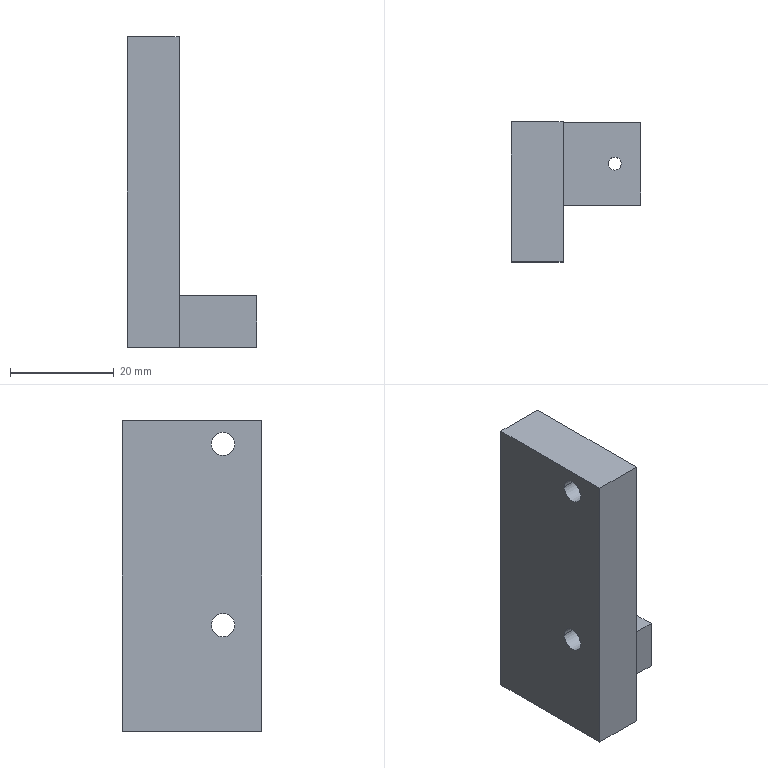Component | SolidWorks | F-YBExport-1-1_LSDH-6-026-1 | 1 solid | 21 faces | box 25 x 27 x 60 mm | volume 17917 mm3 | plane 11 | cylinder 10 | commonest cylinder face diameters 8 x4 4.5 x4 2.5 x2
build123d program:
from build123d import *

# Parameters (mm, degrees)
SKETCH1_W                                            = 60
SKETCH1_H                                            = 10
BOSS_EXTRUDE1_DEPTH                                  = 27
SKETCH2_W                                            = 10
SKETCH2_H                                            = 27
BOSS_EXTRUDE2_DEPTH                                  = 25
HOLE_SIZE_ACCORDING_TO_THE_TYPE_OF_HEX_S_D           = 4.5
HOLE_SIZE_ACCORDING_TO_THE_TYPE_OF_HEX_S_CBORE_D     = 8
HOLE_SIZE_ACCORDING_TO_THE_TYPE_OF_HEX_S_CBORE_DEPTH = 4.6
SKETCH5_W                                            = 11
SKETCH5_H                                            = 25
CUT_EXTRUDE1_DEPTH                                   = 73.312
M3_TAPPED_HOLE1_D                                    = 2.5
SKETCH8_W                                            = 16
SKETCH8_H                                            = 10
CUT_EXTRUDE2_DEPTH                                   = 65.257


with BuildPart() as part:
    # Sketch1 → Boss-Extrude1 (new body)
    with BuildSketch(Plane.XY):
        Rectangle(SKETCH1_W, SKETCH1_H)
    extrude(amount=BOSS_EXTRUDE1_DEPTH)

    # Sketch2 → Boss-Extrude2 (add)
    with BuildSketch(Plane.XZ.offset(5)):
        with Locations((25, 13.5)):
            Rectangle(SKETCH2_W, SKETCH2_H)
    extrude(amount=BOSS_EXTRUDE2_DEPTH)

    # Hole size according to the type of hex s (through all)
    with Locations(Plane(origin=(-25.5, -5, 7.5), x_dir=(0, 0, -1), z_dir=(0, -1, 0))):
        with Locations((0, 0), (0, 35)):
            CounterBoreHole(HOLE_SIZE_ACCORDING_TO_THE_TYPE_OF_HEX_S_D / 2, HOLE_SIZE_ACCORDING_TO_THE_TYPE_OF_HEX_S_CBORE_D / 2, HOLE_SIZE_ACCORDING_TO_THE_TYPE_OF_HEX_S_CBORE_DEPTH)

    # Sketch5 → Cut-Extrude1 (cut, through all)
    with BuildSketch(Plane(origin=(30, 0, 0), x_dir=(0, 0, -1), z_dir=(1, 0, 0))):
        with Locations((-5.5, -17.5)):
            Rectangle(SKETCH5_W, SKETCH5_H)
    extrude(amount=-CUT_EXTRUDE1_DEPTH, mode=Mode.SUBTRACT)

    # M3 Tapped Hole1 (through all)
    with Locations(Plane(origin=(20, -15, 19), x_dir=(0, 0, -1), z_dir=(-1, 0, 0))):
        with Locations((0, 0), (0, 10)):
            Hole(M3_TAPPED_HOLE1_D / 2)

    # Sketch8 → Cut-Extrude2 (cut, through all)
    with BuildSketch(Plane.ZY.offset(-20)):
        with Locations((19, -25)):
            Rectangle(SKETCH8_W, SKETCH8_H)
    extrude(amount=-CUT_EXTRUDE2_DEPTH, mode=Mode.SUBTRACT)


solid = part.part

# Placed as in the assembly
solid = solid.moved(Location((406.305, 356.175, 167.979), (-90, 0, 90)))
STEP:
#1=COLOUR_RGB('',0.7922,0.8196,0.9333);
#2=FILL_AREA_STYLE_COLOUR('',#1);
#3=FILL_AREA_STYLE('',(#2));
#4=SURFACE_STYLE_FILL_AREA(#3);
#5=SURFACE_SIDE_STYLE('',(#4));
#6=SURFACE_STYLE_USAGE(.BOTH.,#5);
#7=PRESENTATION_STYLE_ASSIGNMENT((#6));
#8=CARTESIAN_POINT('',(16.587,14.721,5.432));
#9=VERTEX_POINT('',#8);
#10=CARTESIAN_POINT('',(16.587,14.82,5.432));
#11=VERTEX_POINT('',#10);
#12=CARTESIAN_POINT('',(16.587,14.771,5.432));
#13=DIRECTION('',(-0.,-0.,1.));
#14=DIRECTION('',(0.,1.,0.));
#15=AXIS2_PLACEMENT_3D('',#12,#13,#14);
#16=CIRCLE('',#15,0.04921);
#17=EDGE_CURVE('',#9,#11,#16,.T.);
#18=ORIENTED_EDGE('',*,*,#17,.F.);
#19=CARTESIAN_POINT('',(16.587,14.721,5.826));
#20=VERTEX_POINT('',#19);
#21=CARTESIAN_POINT('',(16.587,14.721,5.826));
#22=DIRECTION('',(-0.,-0.,1.));
#23=VECTOR('',#22,39.37);
#24=LINE('',#21,#23);
#25=EDGE_CURVE('',#9,#20,#24,.T.);
#26=ORIENTED_EDGE('',*,*,#25,.T.);
#27=CARTESIAN_POINT('',(16.587,14.82,5.826));
#28=VERTEX_POINT('',#27);
#29=CARTESIAN_POINT('',(16.587,14.771,5.826));
#30=DIRECTION('',(-0.,-0.,1.));
#31=DIRECTION('',(0.,1.,0.));
#32=AXIS2_PLACEMENT_3D('',#29,#30,#31);
#33=CIRCLE('',#32,0.04921);
#34=EDGE_CURVE('',#20,#28,#33,.T.);
#35=ORIENTED_EDGE('',*,*,#34,.T.);
#36=CARTESIAN_POINT('',(16.587,14.82,5.826));
#37=DIRECTION('',(-0.,-0.,1.));
#38=VECTOR('',#37,39.37);
#39=LINE('',#36,#38);
#40=EDGE_CURVE('',#11,#28,#39,.T.);
#41=ORIENTED_EDGE('',*,*,#40,.F.);
#42=EDGE_LOOP('',(#18,#26,#35,#41));
#43=FACE_OUTER_BOUND('',#42,.T.);
#44=CARTESIAN_POINT('',(16.587,14.771,5.826));
#45=DIRECTION('',(-0.,-0.,1.));
#46=DIRECTION('',(0.,1.,0.));
#47=AXIS2_PLACEMENT_3D('',#44,#45,#46);
#48=CYLINDRICAL_SURFACE('',#47,0.04921);
#49=ADVANCED_FACE('',(#43),#48,.F.);
#50=CARTESIAN_POINT('',(16.012,14.475,7.617));
#51=VERTEX_POINT('',#50);
#52=CARTESIAN_POINT('',(16.012,14.16,7.617));
#53=VERTEX_POINT('',#52);
#54=CARTESIAN_POINT('',(16.012,14.318,7.617));
#55=DIRECTION('',(1.,0.,0.));
#56=DIRECTION('',(0.,-1.,0.));
#57=AXIS2_PLACEMENT_3D('',#54,#55,#56);
#58=CIRCLE('',#57,0.1575);
#59=EDGE_CURVE('',#51,#53,#58,.T.);
#60=ORIENTED_EDGE('',*,*,#59,.F.);
#61=CARTESIAN_POINT('',(16.193,14.475,7.617));
#62=VERTEX_POINT('',#61);
#63=CARTESIAN_POINT('',(16.193,14.475,7.617));
#64=DIRECTION('',(1.,0.,0.));
#65=VECTOR('',#64,39.37);
#66=LINE('',#63,#65);
#67=EDGE_CURVE('',#51,#62,#66,.T.);
#68=ORIENTED_EDGE('',*,*,#67,.T.);
#69=CARTESIAN_POINT('',(16.193,14.16,7.617));
#70=VERTEX_POINT('',#69);
#71=CARTESIAN_POINT('',(16.193,14.318,7.617));
#72=DIRECTION('',(1.,0.,0.));
#73=DIRECTION('',(0.,-1.,0.));
#74=AXIS2_PLACEMENT_3D('',#71,#72,#73);
#75=CIRCLE('',#74,0.1575);
#76=EDGE_CURVE('',#62,#70,#75,.T.);
#77=ORIENTED_EDGE('',*,*,#76,.T.);
#78=CARTESIAN_POINT('',(16.193,14.16,7.617));
#79=DIRECTION('',(1.,0.,0.));
#80=VECTOR('',#79,39.37);
#81=LINE('',#78,#80);
#82=EDGE_CURVE('',#53,#70,#81,.T.);
#83=ORIENTED_EDGE('',*,*,#82,.F.);
#84=EDGE_LOOP('',(#60,#68,#77,#83));
#85=FACE_OUTER_BOUND('',#84,.T.);
#86=CARTESIAN_POINT('',(16.193,14.318,7.617));
#87=DIRECTION('',(1.,0.,0.));
#88=DIRECTION('',(0.,-1.,0.));
#89=AXIS2_PLACEMENT_3D('',#86,#87,#88);
#90=CYLINDRICAL_SURFACE('',#89,0.1575);
#91=ADVANCED_FACE('',(#85),#90,.F.);
#92=CARTESIAN_POINT('',(15.799,14.407,7.617));
#93=VERTEX_POINT('',#92);
#94=CARTESIAN_POINT('',(15.799,14.229,7.617));
#95=VERTEX_POINT('',#94);
#96=CARTESIAN_POINT('',(15.799,14.318,7.617));
#97=DIRECTION('',(1.,0.,0.));
#98=DIRECTION('',(0.,-1.,0.));
#99=AXIS2_PLACEMENT_3D('',#96,#97,#98);
#100=CIRCLE('',#99,0.08858);
#101=EDGE_CURVE('',#93,#95,#100,.T.);
#102=ORIENTED_EDGE('',*,*,#101,.F.);
#103=CARTESIAN_POINT('',(16.012,14.407,7.617));
#104=VERTEX_POINT('',#103);
#105=CARTESIAN_POINT('',(16.193,14.407,7.617));
#106=DIRECTION('',(1.,0.,0.));
#107=VECTOR('',#106,39.37);
#108=LINE('',#105,#107);
#109=EDGE_CURVE('',#93,#104,#108,.T.);
#110=ORIENTED_EDGE('',*,*,#109,.T.);
#111=CARTESIAN_POINT('',(16.012,14.229,7.617));
#112=VERTEX_POINT('',#111);
#113=CARTESIAN_POINT('',(16.012,14.318,7.617));
#114=DIRECTION('',(1.,0.,0.));
#115=DIRECTION('',(0.,-1.,0.));
#116=AXIS2_PLACEMENT_3D('',#113,#114,#115);
#117=CIRCLE('',#116,0.08858);
#118=EDGE_CURVE('',#104,#112,#117,.T.);
#119=ORIENTED_EDGE('',*,*,#118,.T.);
#120=CARTESIAN_POINT('',(16.193,14.229,7.617));
#121=DIRECTION('',(1.,0.,0.));
#122=VECTOR('',#121,39.37);
#123=LINE('',#120,#122);
#124=EDGE_CURVE('',#95,#112,#123,.T.);
#125=ORIENTED_EDGE('',*,*,#124,.F.);
#126=EDGE_LOOP('',(#102,#110,#119,#125));
#127=FACE_OUTER_BOUND('',#126,.T.);
#128=CARTESIAN_POINT('',(16.193,14.318,7.617));
#129=DIRECTION('',(1.,0.,0.));
#130=DIRECTION('',(0.,-1.,0.));
#131=AXIS2_PLACEMENT_3D('',#128,#129,#130);
#132=CYLINDRICAL_SURFACE('',#131,0.08858);
#133=ADVANCED_FACE('',(#127),#132,.F.);
#134=CARTESIAN_POINT('',(16.012,14.475,6.239));
#135=VERTEX_POINT('',#134);
#136=CARTESIAN_POINT('',(16.012,14.16,6.239));
#137=VERTEX_POINT('',#136);
#138=CARTESIAN_POINT('',(16.012,14.318,6.239));
#139=DIRECTION('',(1.,0.,0.));
#140=DIRECTION('',(0.,-1.,0.));
#141=AXIS2_PLACEMENT_3D('',#138,#139,#140);
#142=CIRCLE('',#141,0.1575);
#143=EDGE_CURVE('',#135,#137,#142,.T.);
#144=ORIENTED_EDGE('',*,*,#143,.F.);
#145=CARTESIAN_POINT('',(16.193,14.475,6.239));
#146=VERTEX_POINT('',#145);
#147=CARTESIAN_POINT('',(16.193,14.475,6.239));
#148=DIRECTION('',(1.,0.,0.));
#149=VECTOR('',#148,39.37);
#150=LINE('',#147,#149);
#151=EDGE_CURVE('',#135,#146,#150,.T.);
#152=ORIENTED_EDGE('',*,*,#151,.T.);
#153=CARTESIAN_POINT('',(16.193,14.16,6.239));
#154=VERTEX_POINT('',#153);
#155=CARTESIAN_POINT('',(16.193,14.318,6.239));
#156=DIRECTION('',(1.,0.,0.));
#157=DIRECTION('',(0.,-1.,0.));
#158=AXIS2_PLACEMENT_3D('',#155,#156,#157);
#159=CIRCLE('',#158,0.1575);
#160=EDGE_CURVE('',#146,#154,#159,.T.);
#161=ORIENTED_EDGE('',*,*,#160,.T.);
#162=CARTESIAN_POINT('',(16.193,14.16,6.239));
#163=DIRECTION('',(1.,0.,0.));
#164=VECTOR('',#163,39.37);
#165=LINE('',#162,#164);
#166=EDGE_CURVE('',#137,#154,#165,.T.);
#167=ORIENTED_EDGE('',*,*,#166,.F.);
#168=EDGE_LOOP('',(#144,#152,#161,#167));
#169=FACE_OUTER_BOUND('',#168,.T.);
#170=CARTESIAN_POINT('',(16.193,14.318,6.239));
#171=DIRECTION('',(1.,0.,0.));
#172=DIRECTION('',(0.,-1.,0.));
#173=AXIS2_PLACEMENT_3D('',#170,#171,#172);
#174=CYLINDRICAL_SURFACE('',#173,0.1575);
#175=ADVANCED_FACE('',(#169),#174,.F.);
#176=CARTESIAN_POINT('',(15.799,14.407,6.239));
#177=VERTEX_POINT('',#176);
#178=CARTESIAN_POINT('',(15.799,14.229,6.239));
#179=VERTEX_POINT('',#178);
#180=CARTESIAN_POINT('',(15.799,14.318,6.239));
#181=DIRECTION('',(1.,0.,0.));
#182=DIRECTION('',(0.,-1.,0.));
#183=AXIS2_PLACEMENT_3D('',#180,#181,#182);
#184=CIRCLE('',#183,0.08858);
#185=EDGE_CURVE('',#177,#179,#184,.T.);
#186=ORIENTED_EDGE('',*,*,#185,.F.);
#187=CARTESIAN_POINT('',(16.012,14.407,6.239));
#188=VERTEX_POINT('',#187);
#189=CARTESIAN_POINT('',(16.193,14.407,6.239));
#190=DIRECTION('',(1.,0.,0.));
#191=VECTOR('',#190,39.37);
#192=LINE('',#189,#191);
#193=EDGE_CURVE('',#177,#188,#192,.T.);
#194=ORIENTED_EDGE('',*,*,#193,.T.);
#195=CARTESIAN_POINT('',(16.012,14.229,6.239));
#196=VERTEX_POINT('',#195);
#197=CARTESIAN_POINT('',(16.012,14.318,6.239));
#198=DIRECTION('',(1.,0.,0.));
#199=DIRECTION('',(0.,-1.,0.));
#200=AXIS2_PLACEMENT_3D('',#197,#198,#199);
#201=CIRCLE('',#200,0.08858);
#202=EDGE_CURVE('',#188,#196,#201,.T.);
#203=ORIENTED_EDGE('',*,*,#202,.T.);
#204=CARTESIAN_POINT('',(16.193,14.229,6.239));
#205=DIRECTION('',(1.,0.,0.));
#206=VECTOR('',#205,39.37);
#207=LINE('',#204,#206);
#208=EDGE_CURVE('',#179,#196,#207,.T.);
#209=ORIENTED_EDGE('',*,*,#208,.F.);
#210=EDGE_LOOP('',(#186,#194,#203,#209));
#211=FACE_OUTER_BOUND('',#210,.T.);
#212=CARTESIAN_POINT('',(16.193,14.318,6.239));
#213=DIRECTION('',(1.,0.,0.));
#214=DIRECTION('',(0.,-1.,0.));
#215=AXIS2_PLACEMENT_3D('',#212,#213,#214);
#216=CYLINDRICAL_SURFACE('',#215,0.08858);
#217=ADVANCED_FACE('',(#211),#216,.F.);
#218=CARTESIAN_POINT('',(16.193,14.318,7.617));
#219=DIRECTION('',(1.,0.,0.));
#220=DIRECTION('',(0.,-1.,0.));
#221=AXIS2_PLACEMENT_3D('',#218,#219,#220);
#222=CIRCLE('',#221,0.1575);
#223=EDGE_CURVE('',#70,#62,#222,.T.);
#224=ORIENTED_EDGE('',*,*,#223,.F.);
#225=ORIENTED_EDGE('',*,*,#76,.F.);
#226=EDGE_LOOP('',(#224,#225));
#227=FACE_BOUND('',#226,.T.);
#228=CARTESIAN_POINT('',(16.193,14.318,6.239));
#229=DIRECTION('',(1.,0.,0.));
#230=DIRECTION('',(0.,-1.,0.));
#231=AXIS2_PLACEMENT_3D('',#228,#229,#230);
#232=CIRCLE('',#231,0.1575);
#233=EDGE_CURVE('',#154,#146,#232,.T.);
#234=ORIENTED_EDGE('',*,*,#233,.F.);
#235=ORIENTED_EDGE('',*,*,#160,.F.);
#236=EDGE_LOOP('',(#234,#235));
#237=FACE_BOUND('',#236,.T.);
#238=CARTESIAN_POINT('',(16.193,15.086,7.794));
#239=VERTEX_POINT('',#238);
#240=CARTESIAN_POINT('',(16.193,14.023,7.794));
#241=VERTEX_POINT('',#240);
#242=CARTESIAN_POINT('',(16.193,15.086,7.794));
#243=DIRECTION('',(0.,-1.,0.));
#244=VECTOR('',#243,39.37);
#245=LINE('',#242,#244);
#246=EDGE_CURVE('',#239,#241,#245,.T.);
#247=ORIENTED_EDGE('',*,*,#246,.T.);
#248=CARTESIAN_POINT('',(16.193,14.023,5.432));
#249=VERTEX_POINT('',#248);
#250=CARTESIAN_POINT('',(16.193,14.023,7.794));
#251=DIRECTION('',(0.,0.,-1.));
#252=VECTOR('',#251,39.37);
#253=LINE('',#250,#252);
#254=EDGE_CURVE('',#241,#249,#253,.T.);
#255=ORIENTED_EDGE('',*,*,#254,.T.);
#256=CARTESIAN_POINT('',(16.193,14.456,5.432));
#257=VERTEX_POINT('',#256);
#258=CARTESIAN_POINT('',(16.193,14.023,5.432));
#259=DIRECTION('',(0.,1.,0.));
#260=VECTOR('',#259,39.37);
#261=LINE('',#258,#260);
#262=EDGE_CURVE('',#249,#257,#261,.T.);
#263=ORIENTED_EDGE('',*,*,#262,.T.);
#264=CARTESIAN_POINT('',(16.193,14.456,5.826));
#265=VERTEX_POINT('',#264);
#266=CARTESIAN_POINT('',(16.193,14.456,7.794));
#267=DIRECTION('',(0.,0.,-1.));
#268=VECTOR('',#267,39.37);
#269=LINE('',#266,#268);
#270=EDGE_CURVE('',#265,#257,#269,.T.);
#271=ORIENTED_EDGE('',*,*,#270,.F.);
#272=CARTESIAN_POINT('',(16.193,15.086,5.826));
#273=VERTEX_POINT('',#272);
#274=CARTESIAN_POINT('',(16.193,15.086,5.826));
#275=DIRECTION('',(0.,-1.,-0.));
#276=VECTOR('',#275,39.37);
#277=LINE('',#274,#276);
#278=EDGE_CURVE('',#273,#265,#277,.T.);
#279=ORIENTED_EDGE('',*,*,#278,.F.);
#280=CARTESIAN_POINT('',(16.193,15.086,7.794));
#281=DIRECTION('',(0.,0.,-1.));
#282=VECTOR('',#281,39.37);
#283=LINE('',#280,#282);
#284=EDGE_CURVE('',#239,#273,#283,.T.);
#285=ORIENTED_EDGE('',*,*,#284,.F.);
#286=EDGE_LOOP('',(#247,#255,#263,#271,#279,#285));
#287=FACE_OUTER_BOUND('',#286,.T.);
#288=CARTESIAN_POINT('',(16.193,15.086,7.794));
#289=DIRECTION('',(-1.,0.,-0.));
#290=DIRECTION('',(0.,1.,0.));
#291=AXIS2_PLACEMENT_3D('',#288,#289,#290);
#292=PLANE('',#291);
#293=ADVANCED_FACE('',(#227,#237,#287),#292,.F.);
#294=CARTESIAN_POINT('',(16.587,14.771,5.432));
#295=DIRECTION('',(-0.,-0.,1.));
#296=DIRECTION('',(0.,1.,0.));
#297=AXIS2_PLACEMENT_3D('',#294,#295,#296);
#298=CIRCLE('',#297,0.04921);
#299=EDGE_CURVE('',#11,#9,#298,.T.);
#300=ORIENTED_EDGE('',*,*,#299,.T.);
#301=ORIENTED_EDGE('',*,*,#17,.T.);
#302=EDGE_LOOP('',(#300,#301));
#303=FACE_BOUND('',#302,.T.);
#304=CARTESIAN_POINT('',(16.784,15.086,5.432));
#305=VERTEX_POINT('',#304);
#306=CARTESIAN_POINT('',(15.799,15.086,5.432));
#307=VERTEX_POINT('',#306);
#308=CARTESIAN_POINT('',(15.799,15.086,5.432));
#309=DIRECTION('',(-1.,0.,-0.));
#310=VECTOR('',#309,39.37);
#311=LINE('',#308,#310);
#312=EDGE_CURVE('',#305,#307,#311,.T.);
#313=ORIENTED_EDGE('',*,*,#312,.F.);
#314=CARTESIAN_POINT('',(16.784,14.456,5.432));
#315=VERTEX_POINT('',#314);
#316=CARTESIAN_POINT('',(16.784,14.456,5.432));
#317=DIRECTION('',(0.,-1.,-0.));
#318=VECTOR('',#317,39.37);
#319=LINE('',#316,#318);
#320=EDGE_CURVE('',#305,#315,#319,.T.);
#321=ORIENTED_EDGE('',*,*,#320,.T.);
#322=CARTESIAN_POINT('',(17.177,14.456,5.432));
#323=DIRECTION('',(1.,0.,0.));
#324=VECTOR('',#323,39.37);
#325=LINE('',#322,#324);
#326=EDGE_CURVE('',#257,#315,#325,.T.);
#327=ORIENTED_EDGE('',*,*,#326,.F.);
#328=ORIENTED_EDGE('',*,*,#262,.F.);
#329=CARTESIAN_POINT('',(15.799,14.023,5.432));
#330=VERTEX_POINT('',#329);
#331=CARTESIAN_POINT('',(15.799,14.023,5.432));
#332=DIRECTION('',(-1.,0.,-0.));
#333=VECTOR('',#332,39.37);
#334=LINE('',#331,#333);
#335=EDGE_CURVE('',#249,#330,#334,.T.);
#336=ORIENTED_EDGE('',*,*,#335,.T.);
#337=CARTESIAN_POINT('',(15.799,15.086,5.432));
#338=DIRECTION('',(0.,-1.,0.));
#339=VECTOR('',#338,39.37);
#340=LINE('',#337,#339);
#341=EDGE_CURVE('',#307,#330,#340,.T.);
#342=ORIENTED_EDGE('',*,*,#341,.F.);
#343=EDGE_LOOP('',(#313,#321,#327,#328,#336,#342));
#344=FACE_OUTER_BOUND('',#343,.T.);
#345=CARTESIAN_POINT('',(15.799,15.086,5.432));
#346=DIRECTION('',(-0.,0.,1.));
#347=DIRECTION('',(1.,0.,0.));
#348=AXIS2_PLACEMENT_3D('',#345,#346,#347);
#349=PLANE('',#348);
#350=ADVANCED_FACE('',(#303,#344),#349,.F.);
#351=CARTESIAN_POINT('',(15.799,14.318,7.617));
#352=DIRECTION('',(1.,0.,0.));
#353=DIRECTION('',(0.,-1.,0.));
#354=AXIS2_PLACEMENT_3D('',#351,#352,#353);
#355=CIRCLE('',#354,0.08858);
#356=EDGE_CURVE('',#95,#93,#355,.T.);
#357=ORIENTED_EDGE('',*,*,#356,.T.);
#358=ORIENTED_EDGE('',*,*,#101,.T.);
#359=EDGE_LOOP('',(#357,#358));
#360=FACE_BOUND('',#359,.T.);
#361=CARTESIAN_POINT('',(15.799,14.318,6.239));
#362=DIRECTION('',(1.,0.,0.));
#363=DIRECTION('',(0.,-1.,0.));
#364=AXIS2_PLACEMENT_3D('',#361,#362,#363);
#365=CIRCLE('',#364,0.08858);
#366=EDGE_CURVE('',#179,#177,#365,.T.);
#367=ORIENTED_EDGE('',*,*,#366,.T.);
#368=ORIENTED_EDGE('',*,*,#185,.T.);
#369=EDGE_LOOP('',(#367,#368));
#370=FACE_BOUND('',#369,.T.);
#371=CARTESIAN_POINT('',(15.799,14.023,7.794));
#372=VERTEX_POINT('',#371);
#373=CARTESIAN_POINT('',(15.799,14.023,7.794));
#374=DIRECTION('',(-0.,0.,1.));
#375=VECTOR('',#374,39.37);
#376=LINE('',#373,#375);
#377=EDGE_CURVE('',#330,#372,#376,.T.);
#378=ORIENTED_EDGE('',*,*,#377,.T.);
#379=CARTESIAN_POINT('',(15.799,15.086,7.794));
#380=VERTEX_POINT('',#379);
#381=CARTESIAN_POINT('',(15.799,15.086,7.794));
#382=DIRECTION('',(0.,-1.,0.));
#383=VECTOR('',#382,39.37);
#384=LINE('',#381,#383);
#385=EDGE_CURVE('',#380,#372,#384,.T.);
#386=ORIENTED_EDGE('',*,*,#385,.F.);
#387=CARTESIAN_POINT('',(15.799,15.086,7.794));
#388=DIRECTION('',(-0.,0.,1.));
#389=VECTOR('',#388,39.37);
#390=LINE('',#387,#389);
#391=EDGE_CURVE('',#307,#380,#390,.T.);
#392=ORIENTED_EDGE('',*,*,#391,.F.);
#393=ORIENTED_EDGE('',*,*,#341,.T.);
#394=EDGE_LOOP('',(#378,#386,#392,#393));
#395=FACE_OUTER_BOUND('',#394,.T.);
#396=CARTESIAN_POINT('',(15.799,15.086,7.794));
#397=DIRECTION('',(1.,0.,0.));
#398=DIRECTION('',(0.,-1.,0.));
#399=AXIS2_PLACEMENT_3D('',#396,#397,#398);
#400=PLANE('',#399);
#401=ADVANCED_FACE('',(#360,#370,#395),#400,.F.);
#402=CARTESIAN_POINT('',(15.799,14.023,7.794));
#403=DIRECTION('',(1.,0.,0.));
#404=VECTOR('',#403,39.37);
#405=LINE('',#402,#404);
#406=EDGE_CURVE('',#372,#241,#405,.T.);
#407=ORIENTED_EDGE('',*,*,#406,.T.);
#408=ORIENTED_EDGE('',*,*,#246,.F.);
#409=CARTESIAN_POINT('',(15.799,15.086,7.794));
#410=DIRECTION('',(1.,0.,0.));
#411=VECTOR('',#410,39.37);
#412=LINE('',#409,#411);
#413=EDGE_CURVE('',#380,#239,#412,.T.);
#414=ORIENTED_EDGE('',*,*,#413,.F.);
#415=ORIENTED_EDGE('',*,*,#385,.T.);
#416=EDGE_LOOP('',(#407,#408,#414,#415));
#417=FACE_OUTER_BOUND('',#416,.T.);
#418=CARTESIAN_POINT('',(15.799,15.086,7.794));
#419=DIRECTION('',(0.,0.,-1.));
#420=DIRECTION('',(-1.,0.,-0.));
#421=AXIS2_PLACEMENT_3D('',#418,#419,#420);
#422=PLANE('',#421);
#423=ADVANCED_FACE('',(#417),#422,.F.);
#424=CARTESIAN_POINT('',(16.784,15.086,5.826));
#425=VERTEX_POINT('',#424);
#426=CARTESIAN_POINT('',(16.784,15.086,5.432));
#427=DIRECTION('',(-0.,-0.,1.));
#428=VECTOR('',#427,39.37);
#429=LINE('',#426,#428);
#430=EDGE_CURVE('',#305,#425,#429,.T.);
#431=ORIENTED_EDGE('',*,*,#430,.F.);
#432=ORIENTED_EDGE('',*,*,#312,.T.);
#433=ORIENTED_EDGE('',*,*,#391,.T.);
#434=ORIENTED_EDGE('',*,*,#413,.T.);
#435=ORIENTED_EDGE('',*,*,#284,.T.);
#436=CARTESIAN_POINT('',(17.177,15.086,5.826));
#437=DIRECTION('',(-1.,0.,-0.));
#438=VECTOR('',#437,39.37);
#439=LINE('',#436,#438);
#440=EDGE_CURVE('',#425,#273,#439,.T.);
#441=ORIENTED_EDGE('',*,*,#440,.F.);
#442=EDGE_LOOP('',(#431,#432,#433,#434,#435,#441));
#443=FACE_OUTER_BOUND('',#442,.T.);
#444=CARTESIAN_POINT('',(15.996,15.086,6.613));
#445=DIRECTION('',(0.,1.,0.));
#446=DIRECTION('',(0.,0.,-1.));
#447=AXIS2_PLACEMENT_3D('',#444,#445,#446);
#448=PLANE('',#447);
#449=ADVANCED_FACE('',(#443),#448,.T.);
#450=ORIENTED_EDGE('',*,*,#335,.F.);
#451=ORIENTED_EDGE('',*,*,#254,.F.);
#452=ORIENTED_EDGE('',*,*,#406,.F.);
#453=ORIENTED_EDGE('',*,*,#377,.F.);
#454=EDGE_LOOP('',(#450,#451,#452,#453));
#455=FACE_OUTER_BOUND('',#454,.T.);
#456=CARTESIAN_POINT('',(15.996,14.023,6.613));
#457=DIRECTION('',(0.,1.,0.));
#458=DIRECTION('',(0.,0.,-1.));
#459=AXIS2_PLACEMENT_3D('',#456,#457,#458);
#460=PLANE('',#459);
#461=ADVANCED_FACE('',(#455),#460,.F.);
#462=CARTESIAN_POINT('',(16.587,14.771,5.826));
#463=DIRECTION('',(-0.,-0.,1.));
#464=DIRECTION('',(0.,1.,0.));
#465=AXIS2_PLACEMENT_3D('',#462,#463,#464);
#466=CIRCLE('',#465,0.04921);
#467=EDGE_CURVE('',#28,#20,#466,.T.);
#468=ORIENTED_EDGE('',*,*,#467,.F.);
#469=ORIENTED_EDGE('',*,*,#34,.F.);
#470=EDGE_LOOP('',(#468,#469));
#471=FACE_BOUND('',#470,.T.);
#472=CARTESIAN_POINT('',(16.784,14.456,5.826));
#473=VERTEX_POINT('',#472);
#474=CARTESIAN_POINT('',(17.177,14.456,5.826));
#475=DIRECTION('',(1.,0.,0.));
#476=VECTOR('',#475,39.37);
#477=LINE('',#474,#476);
#478=EDGE_CURVE('',#265,#473,#477,.T.);
#479=ORIENTED_EDGE('',*,*,#478,.T.);
#480=CARTESIAN_POINT('',(16.784,14.456,5.826));
#481=DIRECTION('',(0.,-1.,-0.));
#482=VECTOR('',#481,39.37);
#483=LINE('',#480,#482);
#484=EDGE_CURVE('',#425,#473,#483,.T.);
#485=ORIENTED_EDGE('',*,*,#484,.F.);
#486=ORIENTED_EDGE('',*,*,#440,.T.);
#487=ORIENTED_EDGE('',*,*,#278,.T.);
#488=EDGE_LOOP('',(#479,#485,#486,#487));
#489=FACE_OUTER_BOUND('',#488,.T.);
#490=CARTESIAN_POINT('',(17.177,15.086,5.826));
#491=DIRECTION('',(0.,0.,-1.));
#492=DIRECTION('',(0.,-1.,-0.));
#493=AXIS2_PLACEMENT_3D('',#490,#491,#492);
#494=PLANE('',#493);
#495=ADVANCED_FACE('',(#471,#489),#494,.F.);
#496=ORIENTED_EDGE('',*,*,#193,.F.);
#497=ORIENTED_EDGE('',*,*,#366,.F.);
#498=ORIENTED_EDGE('',*,*,#208,.T.);
#499=CARTESIAN_POINT('',(16.012,14.318,6.239));
#500=DIRECTION('',(1.,0.,0.));
#501=DIRECTION('',(0.,-1.,0.));
#502=AXIS2_PLACEMENT_3D('',#499,#500,#501);
#503=CIRCLE('',#502,0.08858);
#504=EDGE_CURVE('',#196,#188,#503,.T.);
#505=ORIENTED_EDGE('',*,*,#504,.T.);
#506=EDGE_LOOP('',(#496,#497,#498,#505));
#507=FACE_OUTER_BOUND('',#506,.T.);
#508=CARTESIAN_POINT('',(16.193,14.318,6.239));
#509=DIRECTION('',(1.,0.,0.));
#510=DIRECTION('',(0.,-1.,0.));
#511=AXIS2_PLACEMENT_3D('',#508,#509,#510);
#512=CYLINDRICAL_SURFACE('',#511,0.08858);
#513=ADVANCED_FACE('',(#507),#512,.F.);
#514=ORIENTED_EDGE('',*,*,#504,.F.);
#515=ORIENTED_EDGE('',*,*,#202,.F.);
#516=EDGE_LOOP('',(#514,#515));
#517=FACE_BOUND('',#516,.T.);
#518=CARTESIAN_POINT('',(16.012,14.318,6.239));
#519=DIRECTION('',(1.,0.,0.));
#520=DIRECTION('',(0.,-1.,0.));
#521=AXIS2_PLACEMENT_3D('',#518,#519,#520);
#522=CIRCLE('',#521,0.1575);
#523=EDGE_CURVE('',#137,#135,#522,.T.);
#524=ORIENTED_EDGE('',*,*,#523,.T.);
#525=ORIENTED_EDGE('',*,*,#143,.T.);
#526=EDGE_LOOP('',(#524,#525));
#527=FACE_OUTER_BOUND('',#526,.T.);
#528=CARTESIAN_POINT('',(16.012,14.318,6.151));
#529=DIRECTION('',(-1.,0.,-0.));
#530=DIRECTION('',(0.,1.,0.));
#531=AXIS2_PLACEMENT_3D('',#528,#529,#530);
#532=PLANE('',#531);
#533=ADVANCED_FACE('',(#517,#527),#532,.F.);
#534=ORIENTED_EDGE('',*,*,#151,.F.);
#535=ORIENTED_EDGE('',*,*,#523,.F.);
#536=ORIENTED_EDGE('',*,*,#166,.T.);
#537=ORIENTED_EDGE('',*,*,#233,.T.);
#538=EDGE_LOOP('',(#534,#535,#536,#537));
#539=FACE_OUTER_BOUND('',#538,.T.);
#540=CARTESIAN_POINT('',(16.193,14.318,6.239));
#541=DIRECTION('',(1.,0.,0.));
#542=DIRECTION('',(0.,-1.,0.));
#543=AXIS2_PLACEMENT_3D('',#540,#541,#542);
#544=CYLINDRICAL_SURFACE('',#543,0.1575);
#545=ADVANCED_FACE('',(#539),#544,.F.);
#546=ORIENTED_EDGE('',*,*,#109,.F.);
#547=ORIENTED_EDGE('',*,*,#356,.F.);
#548=ORIENTED_EDGE('',*,*,#124,.T.);
#549=CARTESIAN_POINT('',(16.012,14.318,7.617));
#550=DIRECTION('',(1.,0.,0.));
#551=DIRECTION('',(0.,-1.,0.));
#552=AXIS2_PLACEMENT_3D('',#549,#550,#551);
#553=CIRCLE('',#552,0.08858);
#554=EDGE_CURVE('',#112,#104,#553,.T.);
#555=ORIENTED_EDGE('',*,*,#554,.T.);
#556=EDGE_LOOP('',(#546,#547,#548,#555));
#557=FACE_OUTER_BOUND('',#556,.T.);
#558=CARTESIAN_POINT('',(16.193,14.318,7.617));
#559=DIRECTION('',(1.,0.,0.));
#560=DIRECTION('',(0.,-1.,0.));
#561=AXIS2_PLACEMENT_3D('',#558,#559,#560);
#562=CYLINDRICAL_SURFACE('',#561,0.08858);
#563=ADVANCED_FACE('',(#557),#562,.F.);
#564=ORIENTED_EDGE('',*,*,#554,.F.);
#565=ORIENTED_EDGE('',*,*,#118,.F.);
#566=EDGE_LOOP('',(#564,#565));
#567=FACE_BOUND('',#566,.T.);
#568=CARTESIAN_POINT('',(16.012,14.318,7.617));
#569=DIRECTION('',(1.,0.,0.));
#570=DIRECTION('',(0.,-1.,0.));
#571=AXIS2_PLACEMENT_3D('',#568,#569,#570);
#572=CIRCLE('',#571,0.1575);
#573=EDGE_CURVE('',#53,#51,#572,.T.);
#574=ORIENTED_EDGE('',*,*,#573,.T.);
#575=ORIENTED_EDGE('',*,*,#59,.T.);
#576=EDGE_LOOP('',(#574,#575));
#577=FACE_OUTER_BOUND('',#576,.T.);
#578=CARTESIAN_POINT('',(16.012,14.318,7.529));
#579=DIRECTION('',(-1.,0.,-0.));
#580=DIRECTION('',(0.,1.,0.));
#581=AXIS2_PLACEMENT_3D('',#578,#579,#580);
#582=PLANE('',#581);
#583=ADVANCED_FACE('',(#567,#577),#582,.F.);
#584=ORIENTED_EDGE('',*,*,#67,.F.);
#585=ORIENTED_EDGE('',*,*,#573,.F.);
#586=ORIENTED_EDGE('',*,*,#82,.T.);
#587=ORIENTED_EDGE('',*,*,#223,.T.);
#588=EDGE_LOOP('',(#584,#585,#586,#587));
#589=FACE_OUTER_BOUND('',#588,.T.);
#590=CARTESIAN_POINT('',(16.193,14.318,7.617));
#591=DIRECTION('',(1.,0.,0.));
#592=DIRECTION('',(0.,-1.,0.));
#593=AXIS2_PLACEMENT_3D('',#590,#591,#592);
#594=CYLINDRICAL_SURFACE('',#593,0.1575);
#595=ADVANCED_FACE('',(#589),#594,.F.);
#596=ORIENTED_EDGE('',*,*,#326,.T.);
#597=CARTESIAN_POINT('',(16.784,14.456,5.432));
#598=DIRECTION('',(-0.,-0.,1.));
#599=VECTOR('',#598,39.37);
#600=LINE('',#597,#599);
#601=EDGE_CURVE('',#315,#473,#600,.T.);
#602=ORIENTED_EDGE('',*,*,#601,.T.);
#603=ORIENTED_EDGE('',*,*,#478,.F.);
#604=ORIENTED_EDGE('',*,*,#270,.T.);
#605=EDGE_LOOP('',(#596,#602,#603,#604));
#606=FACE_OUTER_BOUND('',#605,.T.);
#607=CARTESIAN_POINT('',(17.177,14.456,7.794));
#608=DIRECTION('',(0.,1.,0.));
#609=DIRECTION('',(0.,0.,-1.));
#610=AXIS2_PLACEMENT_3D('',#607,#608,#609);
#611=PLANE('',#610);
#612=ADVANCED_FACE('',(#606),#611,.F.);
#613=ORIENTED_EDGE('',*,*,#25,.F.);
#614=ORIENTED_EDGE('',*,*,#299,.F.);
#615=ORIENTED_EDGE('',*,*,#40,.T.);
#616=ORIENTED_EDGE('',*,*,#467,.T.);
#617=EDGE_LOOP('',(#613,#614,#615,#616));
#618=FACE_OUTER_BOUND('',#617,.T.);
#619=CARTESIAN_POINT('',(16.587,14.771,5.826));
#620=DIRECTION('',(-0.,-0.,1.));
#621=DIRECTION('',(0.,1.,0.));
#622=AXIS2_PLACEMENT_3D('',#619,#620,#621);
#623=CYLINDRICAL_SURFACE('',#622,0.04921);
#624=ADVANCED_FACE('',(#618),#623,.F.);
#625=ORIENTED_EDGE('',*,*,#484,.T.);
#626=ORIENTED_EDGE('',*,*,#601,.F.);
#627=ORIENTED_EDGE('',*,*,#320,.F.);
#628=ORIENTED_EDGE('',*,*,#430,.T.);
#629=EDGE_LOOP('',(#625,#626,#627,#628));
#630=FACE_OUTER_BOUND('',#629,.T.);
#631=CARTESIAN_POINT('',(16.784,14.456,5.432));
#632=DIRECTION('',(-1.,0.,-0.));
#633=DIRECTION('',(0.,1.,0.));
#634=AXIS2_PLACEMENT_3D('',#631,#632,#633);
#635=PLANE('',#634);
#636=ADVANCED_FACE('',(#630),#635,.F.);
#637=CLOSED_SHELL('',(#49,#91,#133,#175,#217,#293,#350,#401,#423,#449,#461,#495,#513,#533,#545,#563,#583,#595,#612,#624,#636));
#638=MANIFOLD_SOLID_BREP('',#637);
#639=STYLED_ITEM('',(#7),#638);
#640=PRESENTATION_LAYER_ASSIGNMENT('','',(#639));
#641=CARTESIAN_POINT('',(0.,0.,0.));
#642=DIRECTION('',(0.,0.,1.));
#643=DIRECTION('',(1.,0.,0.));
#644=AXIS2_PLACEMENT_3D('',#641,#642,#643);
#645=(LENGTH_UNIT()NAMED_UNIT(*)SI_UNIT($,.METRE.));
#646=LENGTH_MEASURE_WITH_UNIT(LENGTH_MEASURE(0.0254),#645);
#647=DIMENSIONAL_EXPONENTS(1.,0.,0.,0.,0.,0.,0.);
#648=(CONVERSION_BASED_UNIT('',#646)LENGTH_UNIT()NAMED_UNIT(#647));
#649=UNCERTAINTY_MEASURE_WITH_UNIT(LENGTH_MEASURE(0.00001),#648,'','');
#650=(NAMED_UNIT(*)PLANE_ANGLE_UNIT()SI_UNIT($,.RADIAN.));
#651=(NAMED_UNIT(*)SI_UNIT($,.STERADIAN.)SOLID_ANGLE_UNIT());
#652=(GEOMETRIC_REPRESENTATION_CONTEXT(3)GLOBAL_UNCERTAINTY_ASSIGNED_CONTEXT((#649))GLOBAL_UNIT_ASSIGNED_CONTEXT((#648,#650,#651))REPRESENTATION_CONTEXT('',''));
#653=ADVANCED_BREP_SHAPE_REPRESENTATION('',(#638,#644),#652);
#654=(LENGTH_UNIT()NAMED_UNIT(*)SI_UNIT($,.METRE.));
#655=LENGTH_MEASURE_WITH_UNIT(LENGTH_MEASURE(0.0254),#654);
#656=DIMENSIONAL_EXPONENTS(1.,0.,0.,0.,0.,0.,0.);
#657=(CONVERSION_BASED_UNIT('',#655)LENGTH_UNIT()NAMED_UNIT(#656));
#658=UNCERTAINTY_MEASURE_WITH_UNIT(LENGTH_MEASURE(0.00001),#657,'','');
#659=(NAMED_UNIT(*)PLANE_ANGLE_UNIT()SI_UNIT($,.RADIAN.));
#660=(NAMED_UNIT(*)SI_UNIT($,.STERADIAN.)SOLID_ANGLE_UNIT());
#661=(GEOMETRIC_REPRESENTATION_CONTEXT(3)GLOBAL_UNCERTAINTY_ASSIGNED_CONTEXT((#658))GLOBAL_UNIT_ASSIGNED_CONTEXT((#657,#659,#660))REPRESENTATION_CONTEXT('',''));
#662=MECHANICAL_DESIGN_GEOMETRIC_PRESENTATION_REPRESENTATION('',(#639),#661);